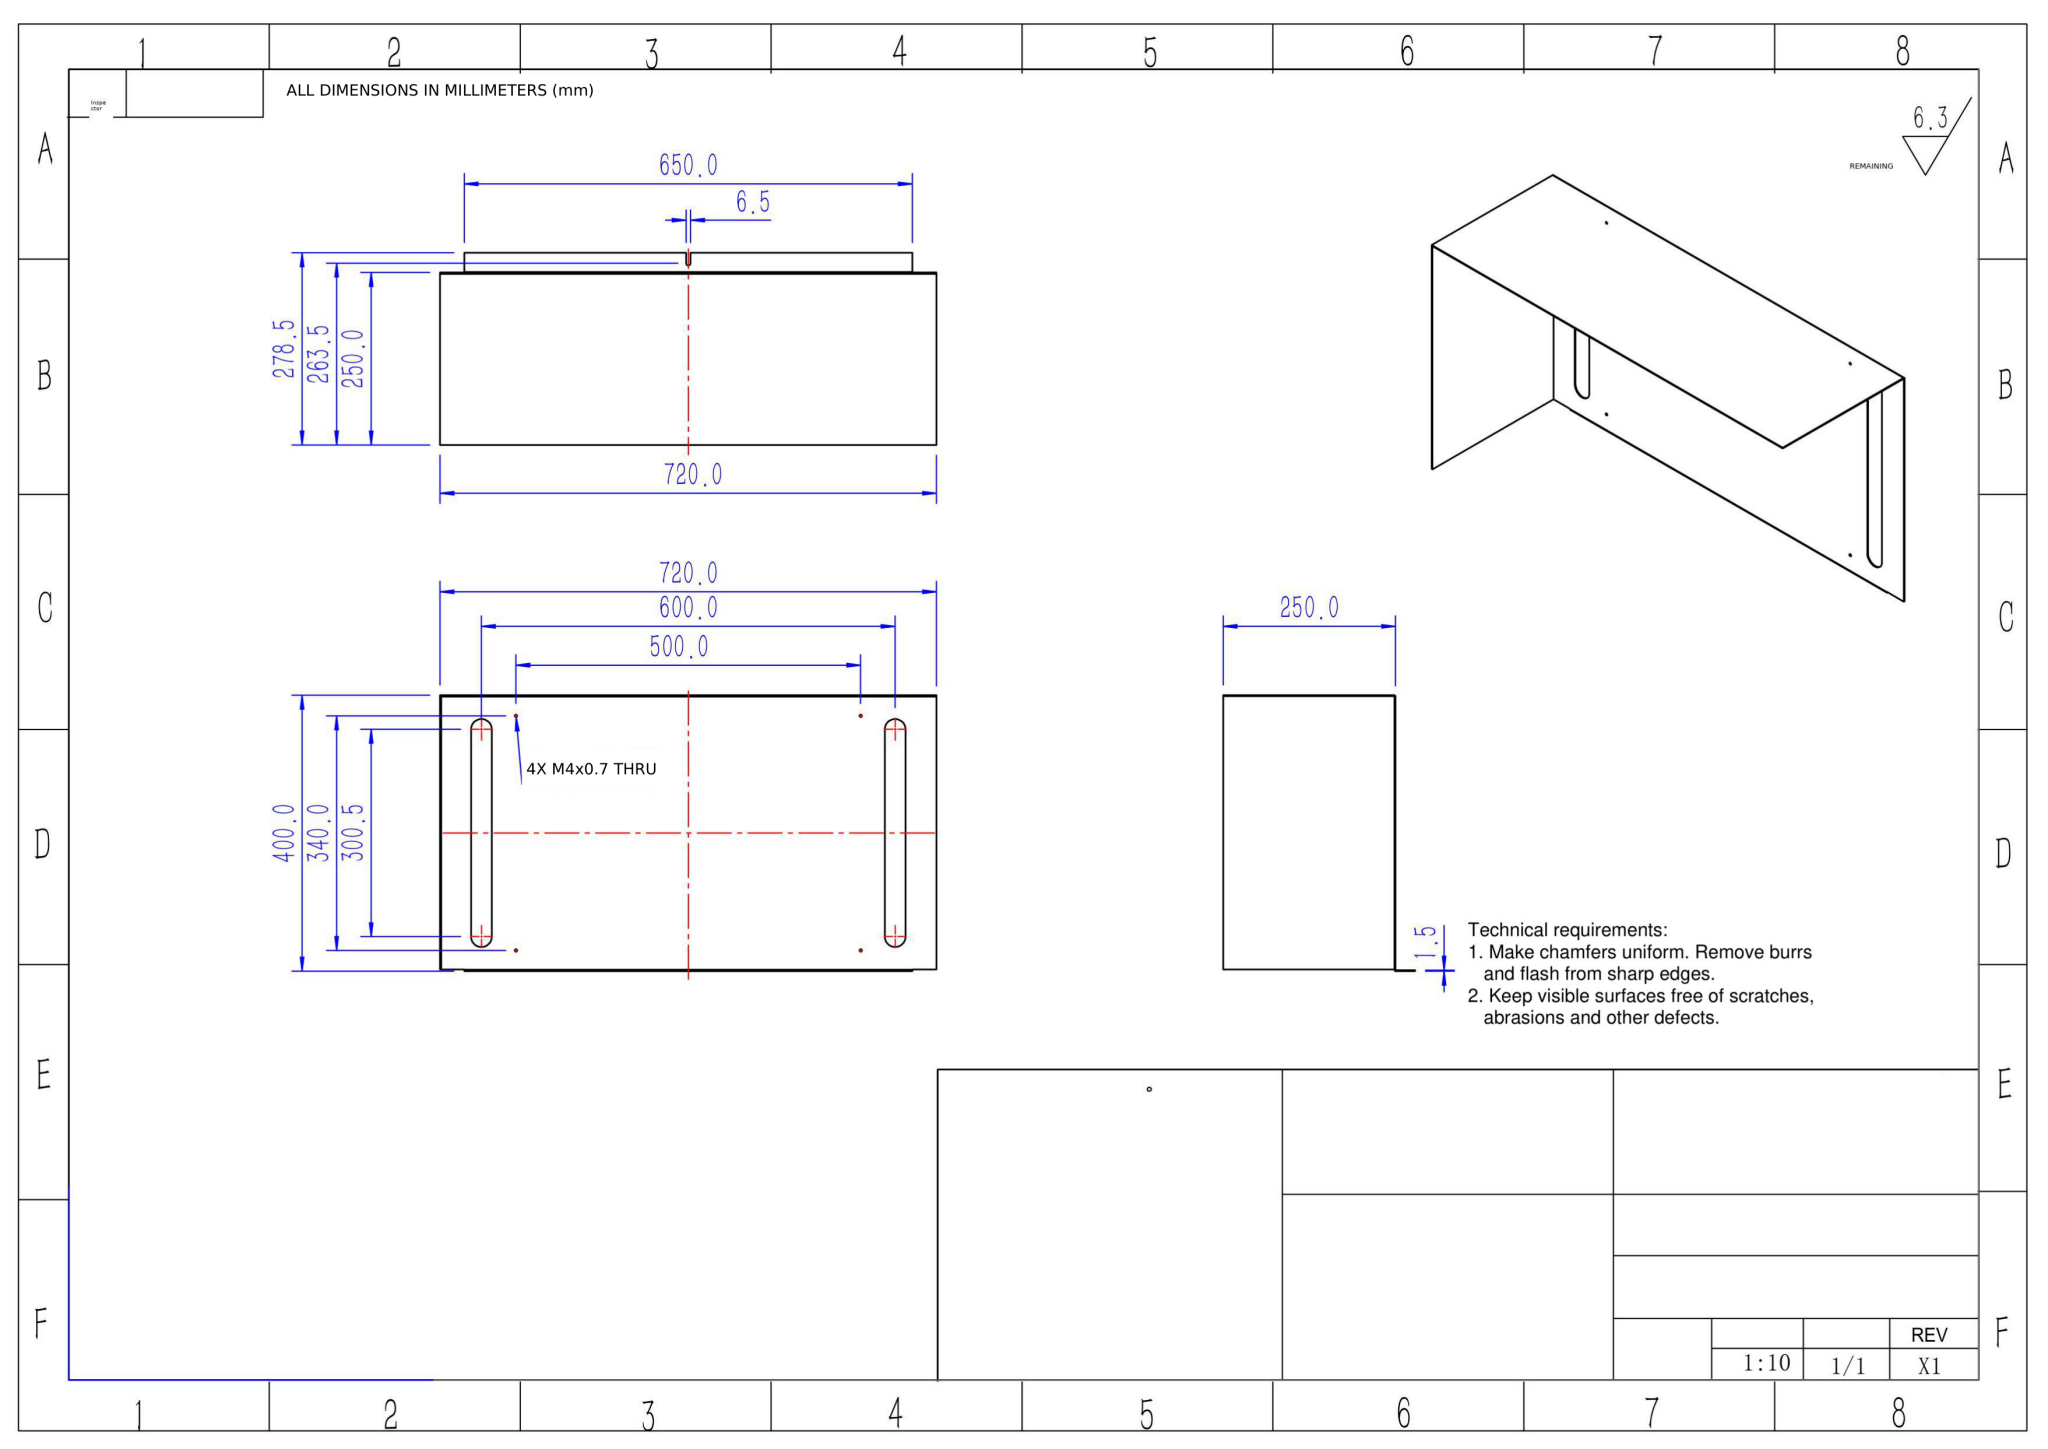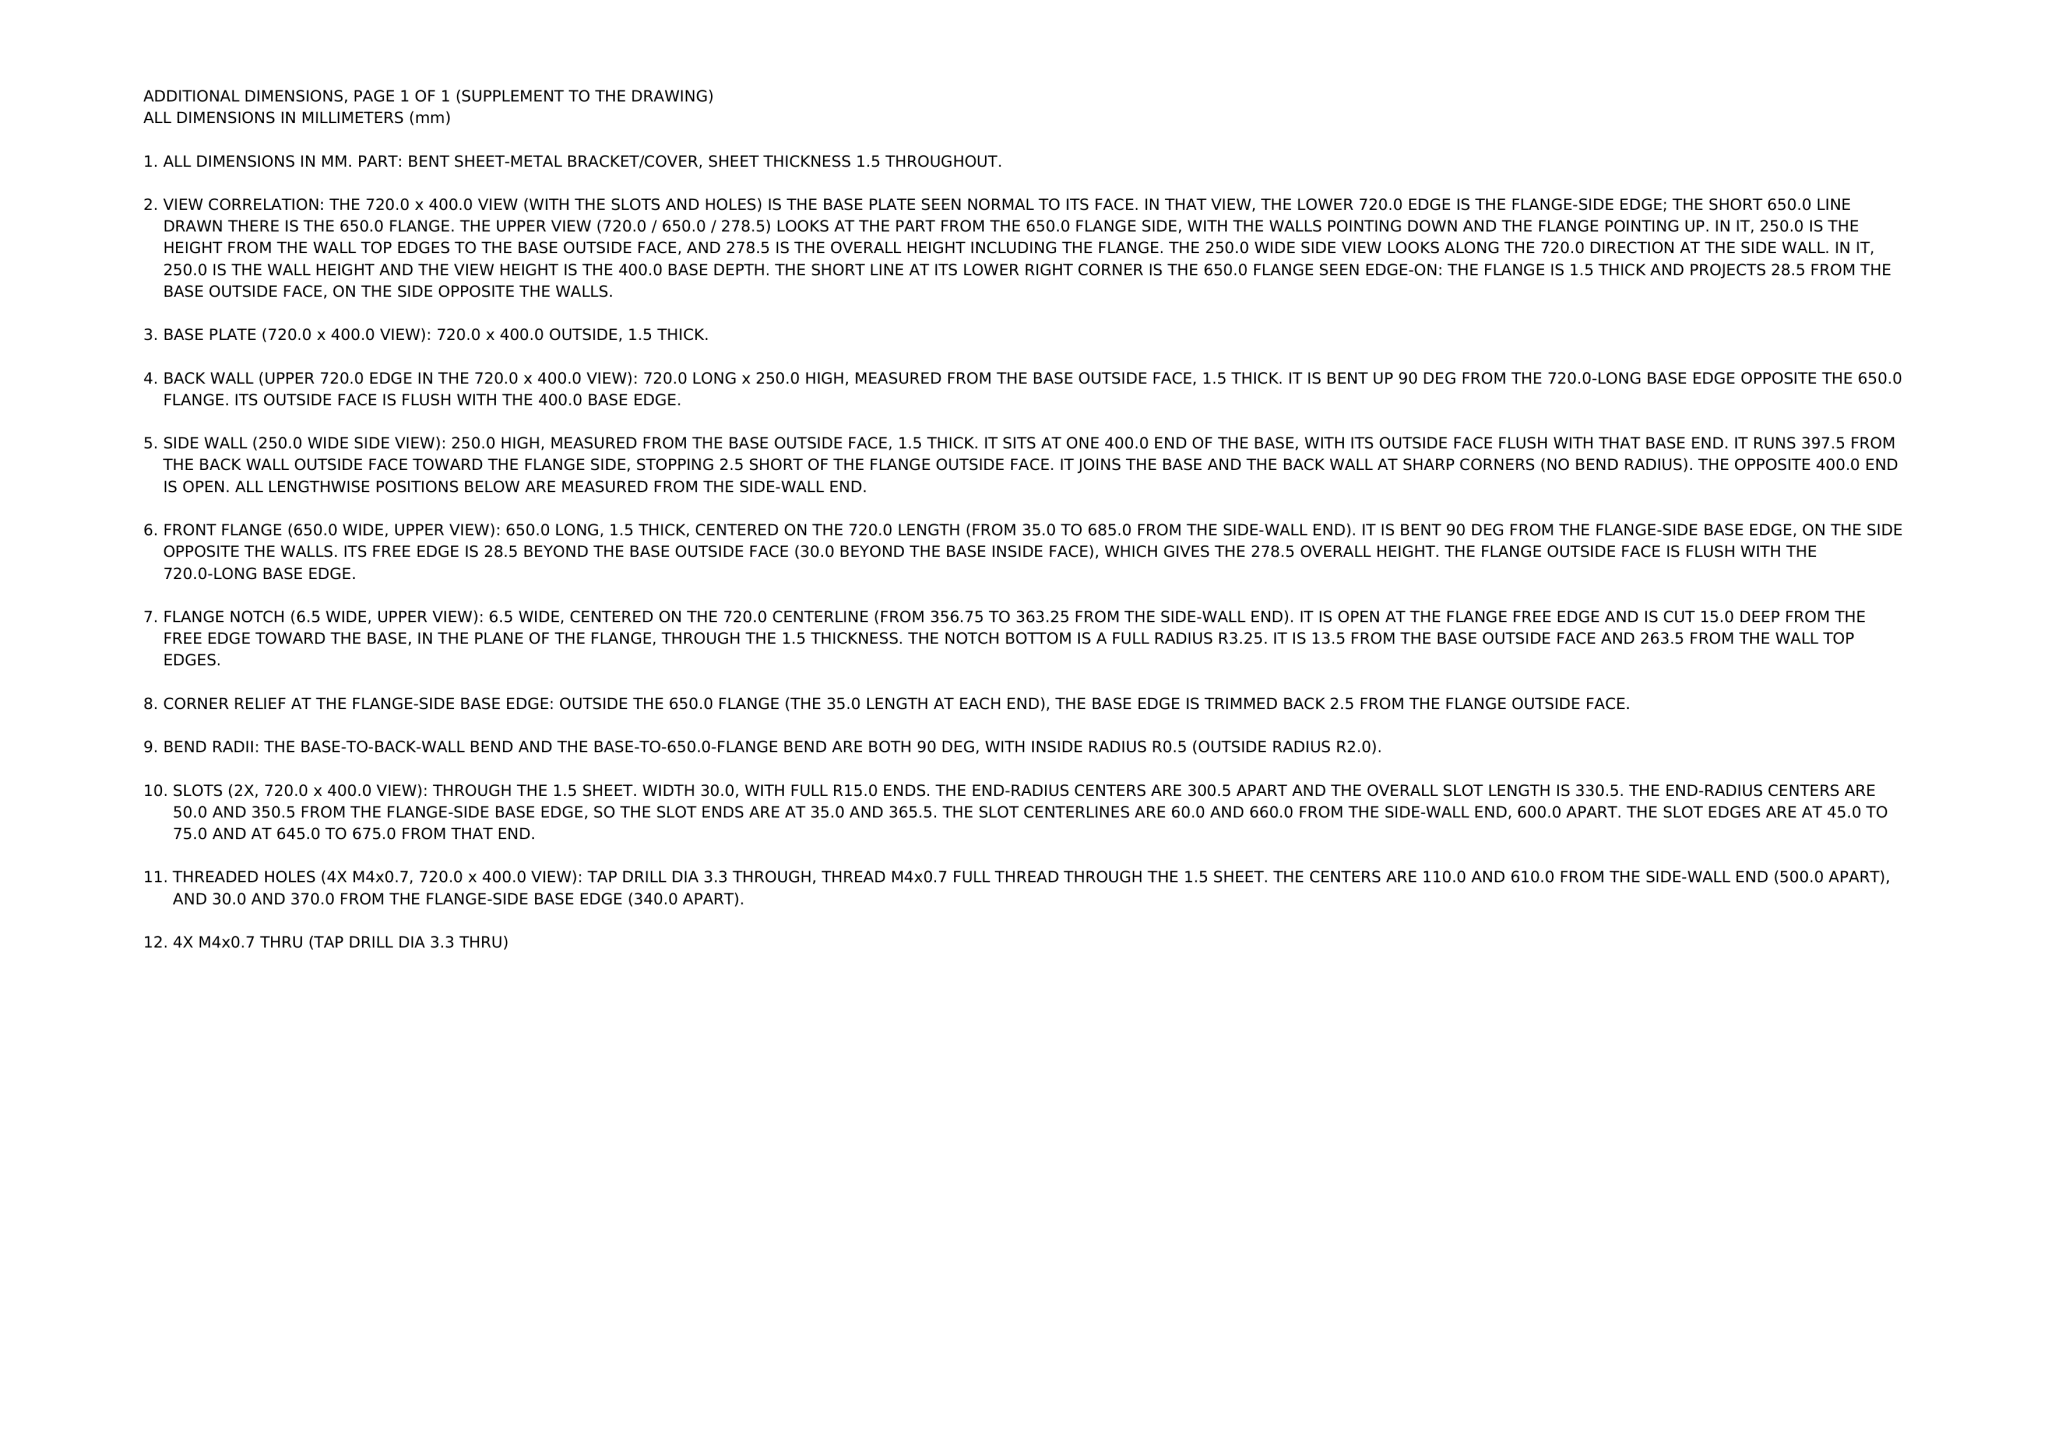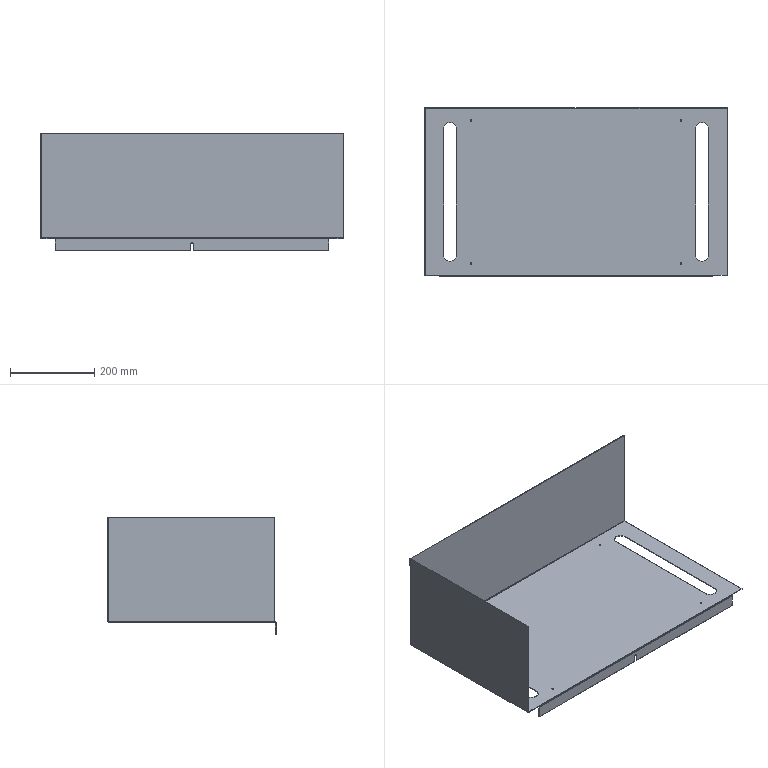Part | NX | mm | 1 solid | 48 faces | box 720 x 400 x 278.5 mm | volume 845023 mm3 | plane 30 | cylinder 18 | commonest cylinder face diameters 3.3 x8 30 x4 6.5 x2 4 x2 1 x2